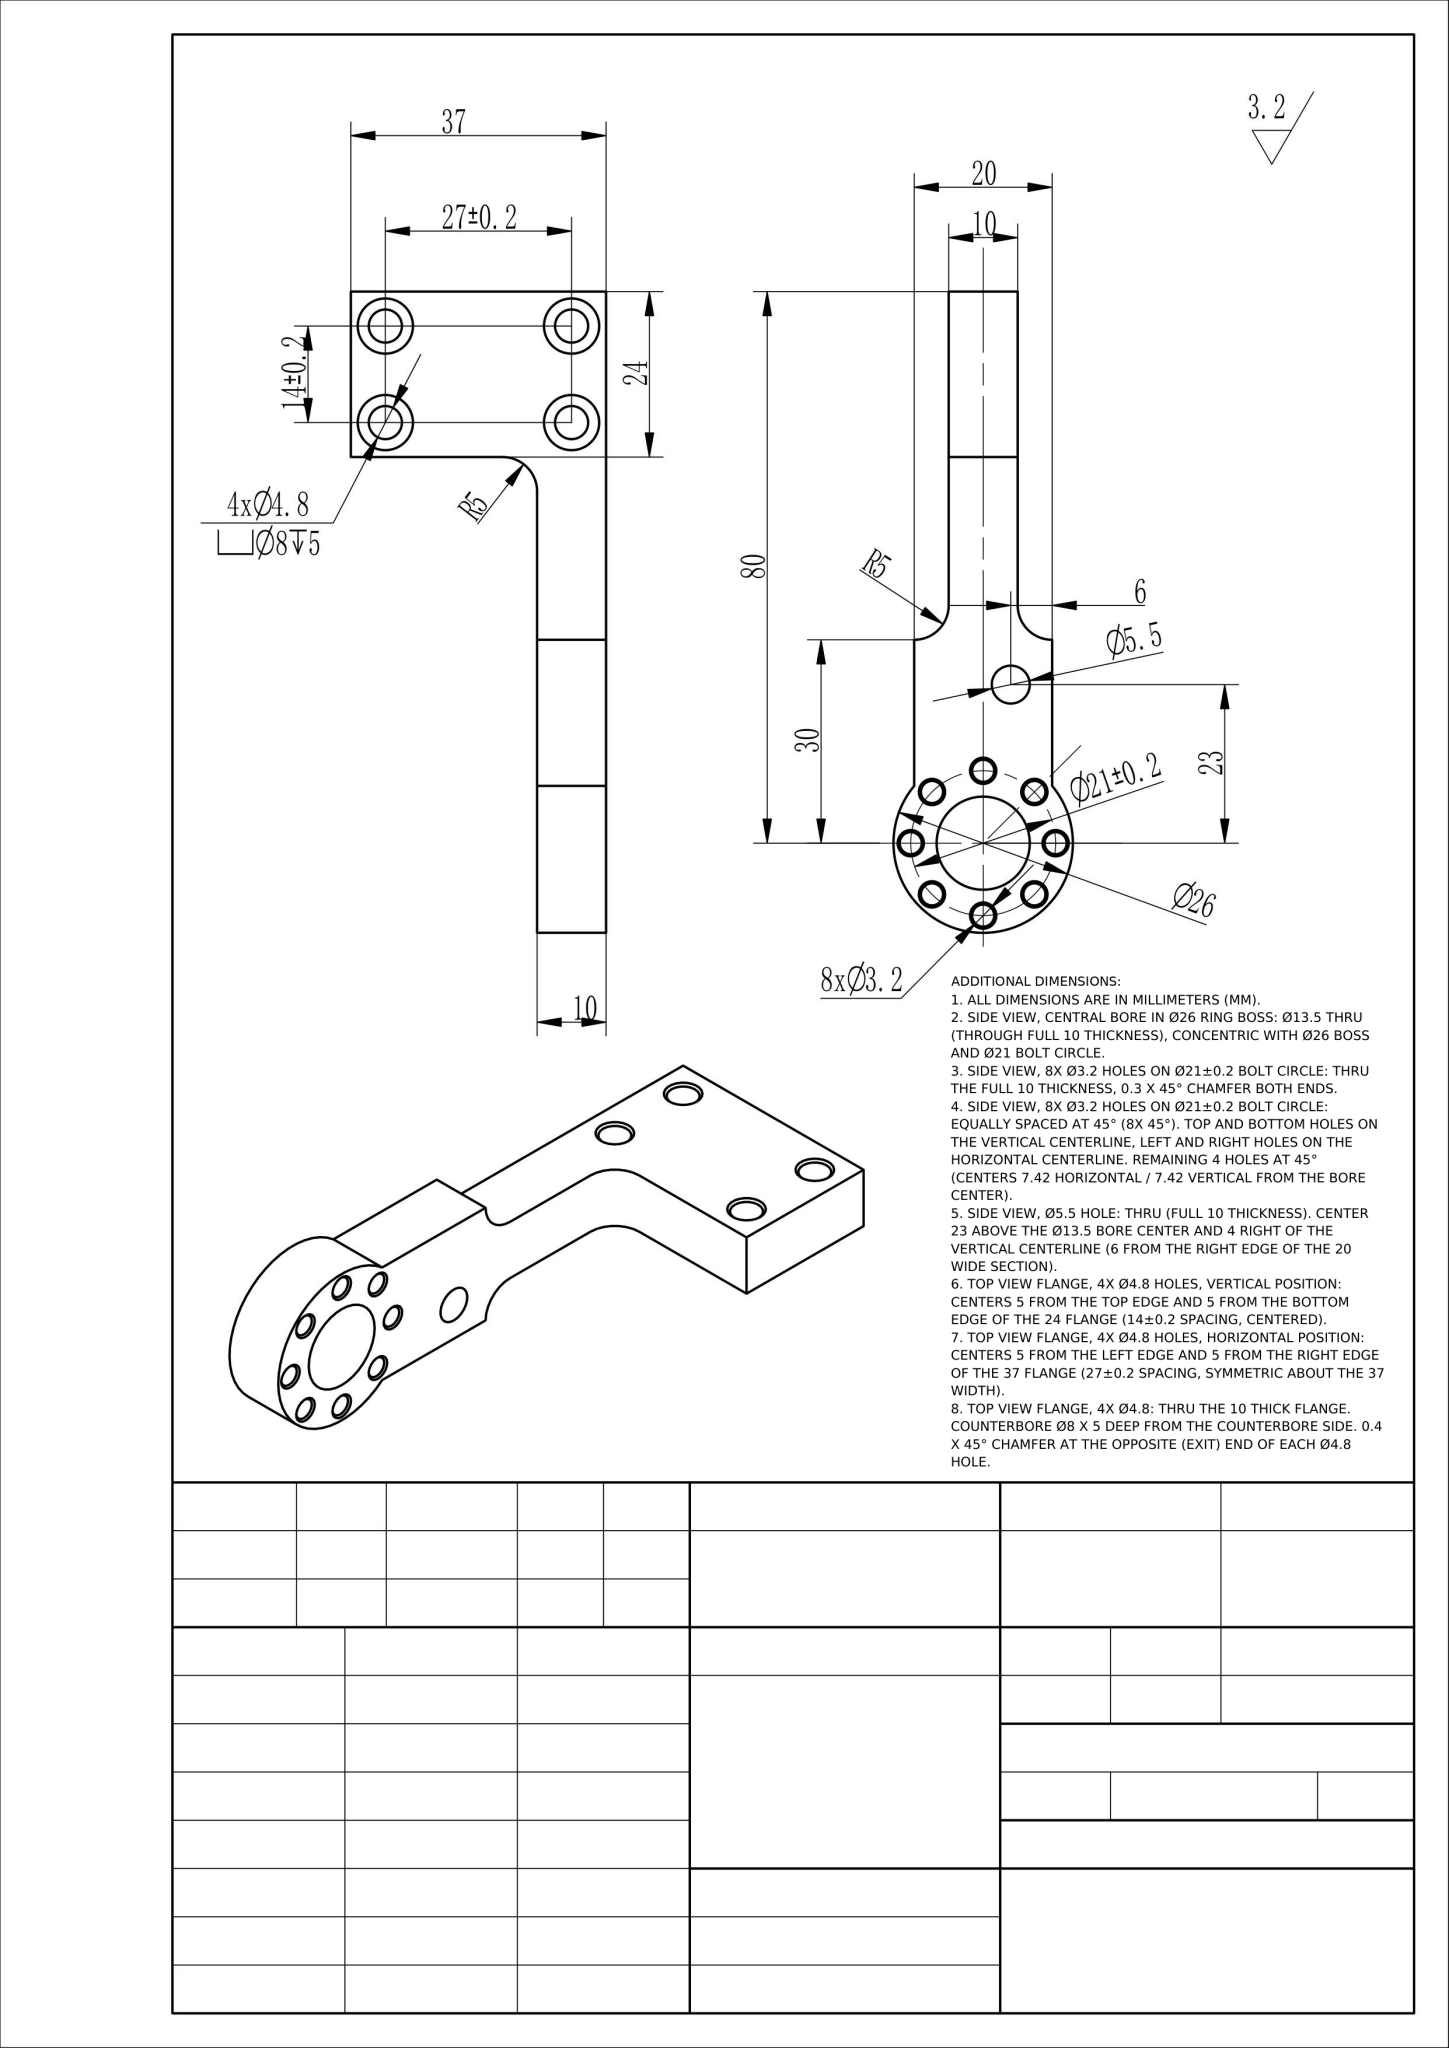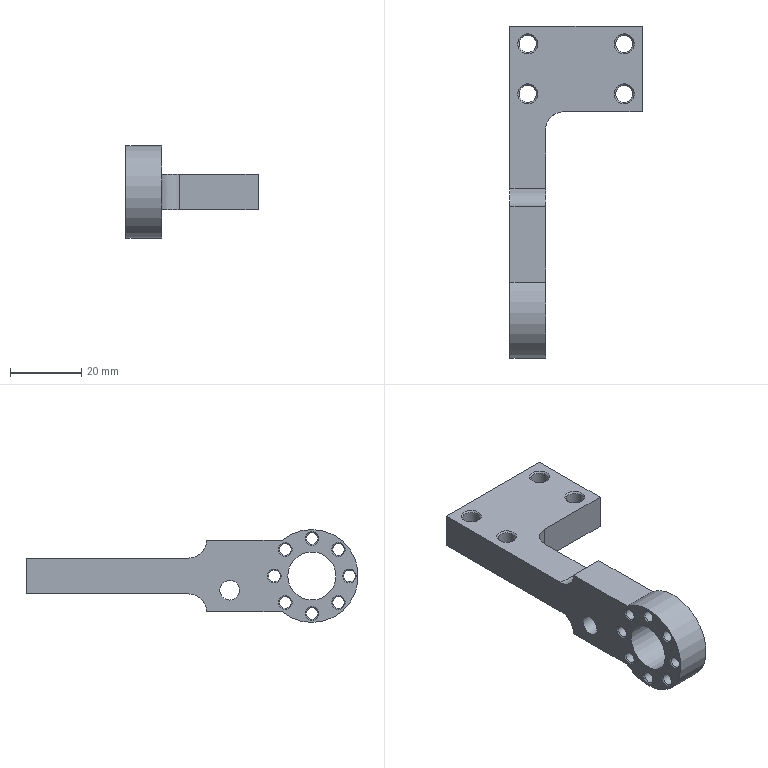Part | NX | mm | 1 solid | 55 faces | box 37 x 93 x 26 mm | volume 16894 mm3 | cylinder 22 | cone 20 | plane 13 | commonest cylinder face diameters 3.2 x8 4.8 x4 8 x4 10 x3 26 x1 13.5 x1 5.5 x1